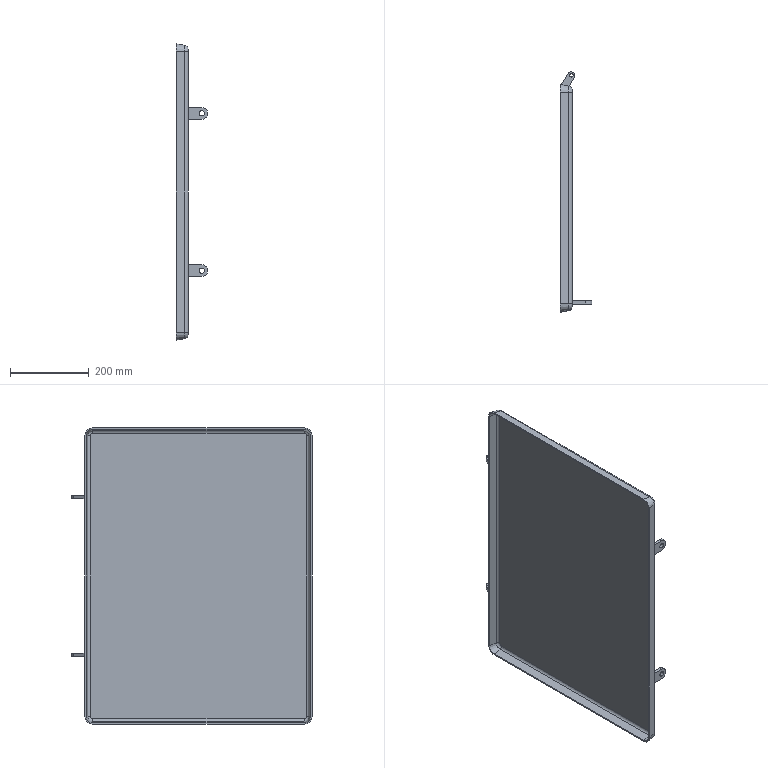Component | SolidWorks | AccessDoor-1 | 1 solid | 66 faces | volume 1492727 mm3 | plane 27 | cylinder 23 | cone 8 | torus 8 | commonest cylinder face diameters 13 x4 9 x4 30 x4 20 x4 14 x4 18 x3